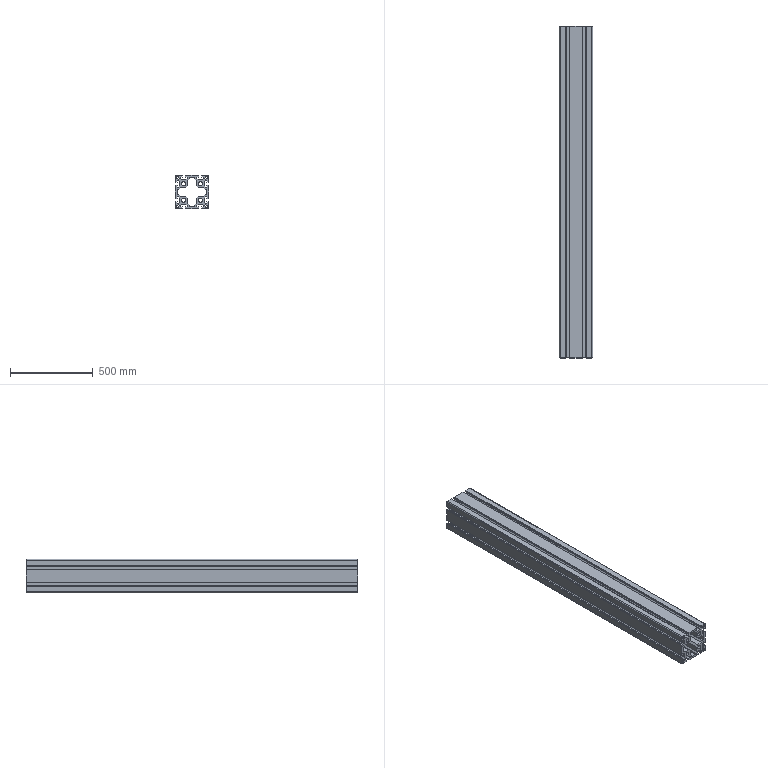Component | SolidWorks | AluminumProfile-1 | 1 solid | 186 faces | box 200 x 2000 x 200 mm | volume 32943809 mm3 | plane 162 | cylinder 24 | commonest cylinder face diameters 12 x12 24 x8 10 x4
build123d program:
from build123d import *

# Parameters (mm, degrees)
SKETCH1_R           = 6
BOSS_EXTRUDE1_DEPTH = 1000
SCALE1_SCALE        = 2


with BuildPart() as part:
    # Sketch1 → Boss-Extrude1 (new body)
    with BuildSketch(Plane(origin=(-310, 0, 0), x_dir=(0, -1, 0), z_dir=(-1, 0, 0))):
        with BuildLine():
            Line((45, 19.9), (45, 14))
            Line((45, 14), (41.657, 14))
            Line((41.657, 14), (37.2, 18.457))
            Line((37.2, 18.457), (37.2, 31.543))
            Line((37.2, 31.543), (41.657, 36))
            Line((41.657, 36), (45, 36))
            Line((45, 36), (45, 30.1))
            Line((45, 30.1), (49, 30.1))
            Line((49, 30.1), (49, 31.1))
            Line((49, 31.1), (50, 31.1))
            Line((50, 31.1), (50, 47.5))
            ThreePointArc((50, 47.5), (49.268, 49.268), (47.5, 50))
            Line((47.5, 50), (31.1, 50))
            Line((31.1, 50), (31.1, 49))
            Line((31.1, 49), (30.1, 49))
            Line((30.1, 49), (30.1, 45))
            Line((30.1, 45), (36, 45))
            Line((36, 45), (36, 41.657))
            Line((36, 41.657), (31.543, 37.2))
            Line((31.543, 37.2), (18.457, 37.2))
            Line((18.457, 37.2), (14, 41.657))
            Line((14, 41.657), (14, 45))
            Line((14, 45), (19.9, 45))
            Line((19.9, 45), (19.9, 49))
            Line((19.9, 49), (18.9, 49))
            Line((18.9, 49), (18.9, 50))
            Line((18.9, 50), (-18.9, 50))
            Line((-18.9, 50), (-18.9, 49))
            Line((-18.9, 49), (-19.9, 49))
            Line((-19.9, 49), (-19.9, 45))
            Line((-19.9, 45), (-14, 45))
            Line((-14, 45), (-14, 41.657))
            Line((-14, 41.657), (-18.457, 37.2))
            Line((-18.457, 37.2), (-31.543, 37.2))
            Line((-31.543, 37.2), (-36, 41.657))
            Line((-36, 41.657), (-36, 45))
            Line((-36, 45), (-30.1, 45))
            Line((-30.1, 45), (-30.1, 49))
            Line((-30.1, 49), (-31.1, 49))
            Line((-31.1, 49), (-31.1, 50))
            Line((-31.1, 50), (-47.5, 50))
            ThreePointArc((-47.5, 50), (-49.268, 49.268), (-50, 47.5))
            Line((-50, 47.5), (-50, 31.1))
            Line((-50, 31.1), (-49, 31.1))
            Line((-49, 31.1), (-49, 30.1))
            Line((-49, 30.1), (-45, 30.1))
            Line((-45, 30.1), (-45, 36))
            Line((-45, 36), (-41.657, 36))
            Line((-41.657, 36), (-37.2, 31.543))
            Line((-37.2, 31.543), (-37.2, 18.457))
            Line((-37.2, 18.457), (-41.657, 14))
            Line((-41.657, 14), (-45, 14))
            Line((-45, 14), (-45, 19.9))
            Line((-45, 19.9), (-49, 19.9))
            Line((-49, 19.9), (-49, 18.9))
            Line((-49, 18.9), (-50, 18.9))
            Line((-50, 18.9), (-50, -18.9))
            Line((-50, -18.9), (-49, -18.9))
            Line((-49, -18.9), (-49, -19.9))
            Line((-49, -19.9), (-45, -19.9))
            Line((-45, -19.9), (-45, -14))
            Line((-45, -14), (-41.657, -14))
            Line((-41.657, -14), (-37.2, -18.457))
            Line((-37.2, -18.457), (-37.2, -31.543))
            Line((-37.2, -31.543), (-41.657, -36))
            Line((-41.657, -36), (-45, -36))
            Line((-45, -36), (-45, -30.1))
            Line((-45, -30.1), (-49, -30.1))
            Line((-49, -30.1), (-49, -31.1))
            Line((-49, -31.1), (-50, -31.1))
            Line((-50, -31.1), (-50, -47.5))
            ThreePointArc((-50, -47.5), (-49.268, -49.268), (-47.5, -50))
            Line((-47.5, -50), (-31.1, -50))
            Line((-31.1, -50), (-31.1, -49))
            Line((-31.1, -49), (-30.1, -49))
            Line((-30.1, -49), (-30.1, -45))
            Line((-30.1, -45), (-36, -45))
            Line((-36, -45), (-36, -41.657))
            Line((-36, -41.657), (-31.543, -37.2))
            Line((-31.543, -37.2), (-18.457, -37.2))
            Line((-18.457, -37.2), (-14, -41.657))
            Line((-14, -41.657), (-14, -45))
            Line((-14, -45), (-19.9, -45))
            Line((-19.9, -45), (-19.9, -49))
            Line((-19.9, -49), (-18.9, -49))
            Line((-18.9, -49), (-18.9, -50))
            Line((-18.9, -50), (18.9, -50))
            Line((18.9, -50), (18.9, -49))
            Line((18.9, -49), (19.9, -49))
            Line((19.9, -49), (19.9, -45))
            Line((19.9, -45), (14, -45))
            Line((14, -45), (14, -41.657))
            Line((14, -41.657), (18.457, -37.2))
            Line((18.457, -37.2), (31.543, -37.2))
            Line((31.543, -37.2), (36, -41.657))
            Line((36, -41.657), (36, -45))
            Line((36, -45), (30.1, -45))
            Line((30.1, -45), (30.1, -49))
            Line((30.1, -49), (31.1, -49))
            Line((31.1, -49), (31.1, -50))
            Line((31.1, -50), (47.5, -50))
            ThreePointArc((47.5, -50), (49.268, -49.268), (50, -47.5))
            Line((50, -47.5), (50, -31.1))
            Line((50, -31.1), (49, -31.1))
            Line((49, -31.1), (49, -30.1))
            Line((49, -30.1), (45, -30.1))
            Line((45, -30.1), (45, -36))
            Line((45, -36), (41.657, -36))
            Line((41.657, -36), (37.2, -31.543))
            Line((37.2, -31.543), (37.2, -18.457))
            Line((37.2, -18.457), (41.657, -14))
            Line((41.657, -14), (45, -14))
            Line((45, -14), (45, -19.9))
            Line((45, -19.9), (49, -19.9))
            Line((49, -19.9), (49, -18.9))
            Line((49, -18.9), (50, -18.9))
            Line((50, -18.9), (50, 18.9))
            Line((50, 18.9), (49, 18.9))
            Line((49, 18.9), (49, 19.9))
            Line((49, 19.9), (45, 19.9))
        make_face()
        with Locations(Location((25, 25, 0), (0, 0, 180))):
            Circle(SKETCH1_R, mode=Mode.SUBTRACT)
        with Locations(Location((25, -25, 0), (0, 0, 180))):
            Circle(SKETCH1_R, mode=Mode.SUBTRACT)
        with Locations(Location((-25, 25, 0), (0, 0, 180))):
            Circle(SKETCH1_R, mode=Mode.SUBTRACT)
        with Locations(Location((-25, -25, 0), (0, 0, 180))):
            Circle(SKETCH1_R, mode=Mode.SUBTRACT)
        with BuildLine():
            Line((38.981, -40.678), (40.678, -38.981))
            Line((40.678, -38.981), (42.904, -41.207))
            ThreePointArc((42.904, -41.207), (46.121, -46.121), (41.207, -42.904))
            Line((41.207, -42.904), (38.981, -40.678))
        make_face(mode=Mode.SUBTRACT)
        with BuildLine():
            Line((-40.678, -38.981), (-38.981, -40.678))
            Line((-38.981, -40.678), (-41.207, -42.904))
            ThreePointArc((-41.207, -42.904), (-46.121, -46.121), (-42.904, -41.207))
            Line((-42.904, -41.207), (-40.678, -38.981))
        make_face(mode=Mode.SUBTRACT)
        Polygon((34.372, 12.8), (39.172, 8), (44, 8), (44, -8), (39.172, -8), (34.372, -12.8), (18.8, -12.8), (12.8, -18.8), (12.8, -34.372), (8, -39.172), (8, -44), (-8, -44), (-8, -39.172), (-12.8, -34.372), (-12.8, -18.8), (-18.8, -12.8), (-34.372, -12.8), (-39.172, -8), (-44, -8), (-44, 8), (-39.172, 8), (-34.372, 12.8), (-18.8, 12.8), (-12.8, 18.8), (-12.8, 34.372), (-8, 39.172), (-8, 44), (8, 44), (8, 39.172), (12.8, 34.372), (12.8, 18.8), (18.8, 12.8), align=None, mode=Mode.SUBTRACT)
        with BuildLine():
            Line((42.904, 41.207), (40.678, 38.981))
            Line((40.678, 38.981), (38.981, 40.678))
            Line((38.981, 40.678), (41.207, 42.904))
            ThreePointArc((41.207, 42.904), (46.121, 46.121), (42.904, 41.207))
        make_face(mode=Mode.SUBTRACT)
        with BuildLine():
            Line((-41.207, 42.904), (-38.981, 40.678))
            Line((-38.981, 40.678), (-40.678, 38.981))
            Line((-40.678, 38.981), (-42.904, 41.207))
            ThreePointArc((-42.904, 41.207), (-46.121, 46.121), (-41.207, 42.904))
        make_face(mode=Mode.SUBTRACT)
    extrude(amount=-BOSS_EXTRUDE1_DEPTH)


with BuildPart() as part_1:
    # Scale1: scaled about (190, 0, -0)
    add(part.part.scale(SCALE1_SCALE).moved(Location((-190, 0, 0))))


solid = part_1.part

# Placed as in the assembly
solid = solid.moved(Location((2286, -221, -255), (0, 0, 90)))